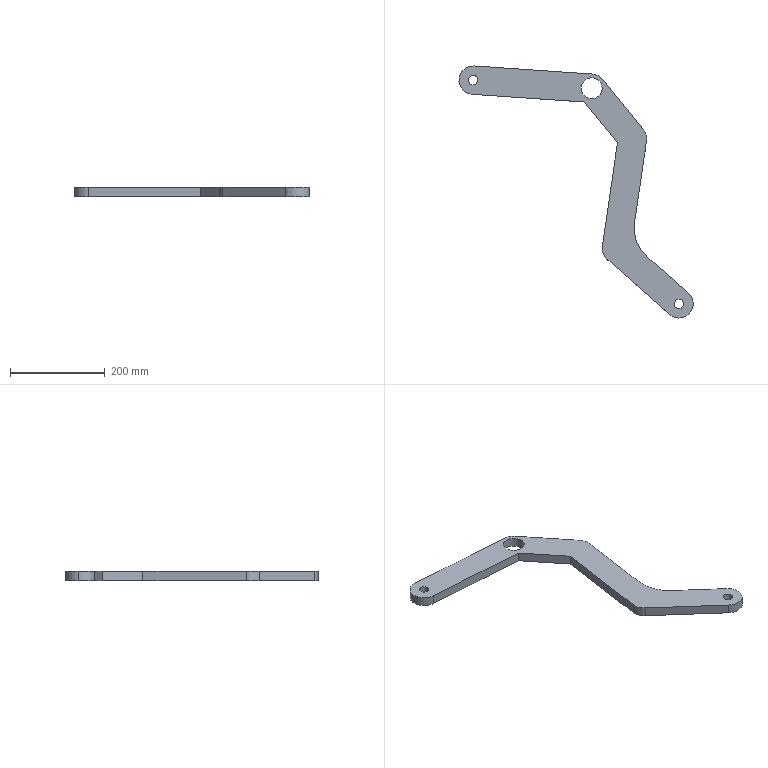Component | SolidWorks | IngotSupportRod-13 | 1 solid | 23 faces | box 494.09 x 531.83 x 20 mm | volume 974379 mm3 | cylinder 13 | plane 10 | commonest cylinder face diameters 60 x6 20 x4 44.189 x2 160 x1 | material 45
build123d program:
from build123d import *

# Parameters (mm, degrees)
SKETCH1_R           = 22.094
SKETCH1_R_2         = 10
BOSS_EXTRUDE1_DEPTH = 20
SKETCH2_R           = 22.094
BOSS_EXTRUDE2_DEPTH = 20
SKETCH3_R           = 10
CUT_EXTRUDE1_DEPTH  = 20


with BuildPart() as part:
    # Sketch1 → Boss-Extrude1 (new body)
    # profile 1 of 3: a face of its own
    with BuildSketch(Plane.XY):
        with BuildLine():
            Line((541.993, 526.894), (441.544, 620.054))
            ThreePointArc((441.544, 620.054), (399.148, 618.458), (400.744, 576.062))
            Line((400.744, 576.062), (491.593, 491.805))
            Line((491.593, 491.805), (491.593, 504.898))
            ThreePointArc((491.593, 504.898), (509.593, 532.394), (541.993, 526.894))
        make_face()
        with Locations((421.144, 598.058)):
            Circle(SKETCH1_R, mode=Mode.SUBTRACT)
    # profile 2 of 3: a face of its own
    with BuildSketch(Plane.XY):
        with BuildLine():
            Line((551.593, 330.656), (551.593, 504.898))
            ThreePointArc((551.593, 504.898), (533.593, 477.403), (501.193, 482.902))
            Line((501.193, 482.902), (491.593, 491.805))
            Line((491.593, 491.805), (491.593, 271.193))
            ThreePointArc((491.593, 271.193), (495.202, 256.927), (505.161, 246.094))
            Line((505.161, 246.094), (652.514, 149.626))
            ThreePointArc((652.514, 149.626), (694.046, 158.294), (685.378, 199.825))
            Line((685.378, 199.825), (587.775, 263.724))
            ThreePointArc((587.775, 263.724), (561.218, 292.613), (551.593, 330.656))
        make_face()
        with Locations((668.946, 174.726)):
            Circle(SKETCH1_R_2, mode=Mode.SUBTRACT)
    # profile 3 of 3: a face of its own
    with BuildSketch(Plane.XY):
        with BuildLine():
            ThreePointArc((551.593, 504.898), (549.089, 516.898), (541.993, 526.894))
            ThreePointArc((541.993, 526.894), (509.593, 532.394), (491.593, 504.898))
            Line((491.593, 504.898), (491.593, 491.805))
            Line((491.593, 491.805), (501.193, 482.902))
            ThreePointArc((501.193, 482.902), (533.593, 477.403), (551.593, 504.898))
        make_face()
    extrude(amount=BOSS_EXTRUDE1_DEPTH)

    # Sketch2 → Boss-Extrude2 (add)
    with BuildSketch(Plane.XY):
        with BuildLine():
            Line((423.445, 568.146), (173.493, 548.919))
            ThreePointArc((173.493, 548.919), (141.281, 576.53), (168.892, 608.742))
            Line((168.892, 608.742), (418.843, 627.97))
            ThreePointArc((418.843, 627.97), (451.056, 600.359), (423.445, 568.146))
        make_face()
        with Locations((421.144, 598.058)):
            Circle(SKETCH2_R, mode=Mode.SUBTRACT)
    extrude(amount=BOSS_EXTRUDE2_DEPTH)

    # Sketch3 → Cut-Extrude1 (cut)
    with BuildSketch(Plane.XY.offset(20)):
        with Locations((171.193, 578.831)):
            Circle(SKETCH3_R)
    extrude(amount=-CUT_EXTRUDE1_DEPTH, mode=Mode.SUBTRACT)


solid = part.part

# Placed as in the assembly
solid = solid.moved(Location((17.945, 67.185, 545), (0, 0, -8.314)))
STEP:
#1=COLOUR_RGB('',0.7922,0.8196,0.9333);
#2=FILL_AREA_STYLE_COLOUR('',#1);
#3=FILL_AREA_STYLE('',(#2));
#4=SURFACE_STYLE_FILL_AREA(#3);
#5=SURFACE_SIDE_STYLE('',(#4));
#6=SURFACE_STYLE_USAGE(.BOTH.,#5);
#7=PRESENTATION_STYLE_ASSIGNMENT((#6));
#8=CARTESIAN_POINT('',(10.281,24.276,21.457));
#9=VERTEX_POINT('',#8);
#10=CARTESIAN_POINT('',(11.06,24.163,21.457));
#11=VERTEX_POINT('',#10);
#12=CARTESIAN_POINT('',(10.671,24.22,21.457));
#13=DIRECTION('',(-0.,0.,1.));
#14=DIRECTION('',(0.9895,-0.1446,0.));
#15=AXIS2_PLACEMENT_3D('',#12,#13,#14);
#16=CIRCLE('',#15,0.3937);
#17=EDGE_CURVE('',#9,#11,#16,.T.);
#18=ORIENTED_EDGE('',*,*,#17,.F.);
#19=CARTESIAN_POINT('',(10.281,24.276,22.244));
#20=VERTEX_POINT('',#19);
#21=CARTESIAN_POINT('',(10.281,24.276,21.457));
#22=DIRECTION('',(-0.,0.,1.));
#23=VECTOR('',#22,39.37);
#24=LINE('',#21,#23);
#25=EDGE_CURVE('',#9,#20,#24,.T.);
#26=ORIENTED_EDGE('',*,*,#25,.T.);
#27=CARTESIAN_POINT('',(11.06,24.163,22.244));
#28=VERTEX_POINT('',#27);
#29=CARTESIAN_POINT('',(10.671,24.22,22.244));
#30=DIRECTION('',(-0.,0.,1.));
#31=DIRECTION('',(0.9895,-0.1446,0.));
#32=AXIS2_PLACEMENT_3D('',#29,#30,#31);
#33=CIRCLE('',#32,0.3937);
#34=EDGE_CURVE('',#20,#28,#33,.T.);
#35=ORIENTED_EDGE('',*,*,#34,.T.);
#36=CARTESIAN_POINT('',(11.06,24.163,21.457));
#37=DIRECTION('',(-0.,0.,1.));
#38=VECTOR('',#37,39.37);
#39=LINE('',#36,#38);
#40=EDGE_CURVE('',#11,#28,#39,.T.);
#41=ORIENTED_EDGE('',*,*,#40,.F.);
#42=EDGE_LOOP('',(#18,#26,#35,#41));
#43=FACE_OUTER_BOUND('',#42,.T.);
#44=CARTESIAN_POINT('',(10.671,24.22,21.457));
#45=DIRECTION('',(-0.,0.,1.));
#46=DIRECTION('',(0.9895,-0.1446,0.));
#47=AXIS2_PLACEMENT_3D('',#44,#45,#46);
#48=CYLINDRICAL_SURFACE('',#47,0.3937);
#49=ADVANCED_FACE('',(#43),#48,.F.);
#50=CARTESIAN_POINT('',(9.502,24.39,22.244));
#51=VERTEX_POINT('',#50);
#52=CARTESIAN_POINT('',(10.59,23.041,22.244));
#53=VERTEX_POINT('',#52);
#54=CARTESIAN_POINT('',(10.671,24.22,22.244));
#55=DIRECTION('',(-0.,0.,1.));
#56=DIRECTION('',(0.9895,-0.1446,0.));
#57=AXIS2_PLACEMENT_3D('',#54,#55,#56);
#58=CIRCLE('',#57,1.181);
#59=EDGE_CURVE('',#51,#53,#58,.T.);
#60=ORIENTED_EDGE('',*,*,#59,.F.);
#61=CARTESIAN_POINT('',(9.502,24.39,21.457));
#62=VERTEX_POINT('',#61);
#63=CARTESIAN_POINT('',(9.502,24.39,22.244));
#64=DIRECTION('',(0.,-0.,-1.));
#65=VECTOR('',#64,39.37);
#66=LINE('',#63,#65);
#67=EDGE_CURVE('',#51,#62,#66,.T.);
#68=ORIENTED_EDGE('',*,*,#67,.T.);
#69=CARTESIAN_POINT('',(10.59,23.041,21.457));
#70=VERTEX_POINT('',#69);
#71=CARTESIAN_POINT('',(10.671,24.22,21.457));
#72=DIRECTION('',(-0.,0.,1.));
#73=DIRECTION('',(0.9895,-0.1446,0.));
#74=AXIS2_PLACEMENT_3D('',#71,#72,#73);
#75=CIRCLE('',#74,1.181);
#76=EDGE_CURVE('',#62,#70,#75,.T.);
#77=ORIENTED_EDGE('',*,*,#76,.T.);
#78=CARTESIAN_POINT('',(10.59,23.041,22.244));
#79=DIRECTION('',(0.,-0.,-1.));
#80=VECTOR('',#79,39.37);
#81=LINE('',#78,#80);
#82=EDGE_CURVE('',#53,#70,#81,.T.);
#83=ORIENTED_EDGE('',*,*,#82,.F.);
#84=EDGE_LOOP('',(#60,#68,#77,#83));
#85=FACE_OUTER_BOUND('',#84,.T.);
#86=CARTESIAN_POINT('',(10.671,24.22,22.244));
#87=DIRECTION('',(0.,-0.,-1.));
#88=DIRECTION('',(-0.9895,0.1446,0.));
#89=AXIS2_PLACEMENT_3D('',#86,#87,#88);
#90=CYLINDRICAL_SURFACE('',#89,1.181);
#91=ADVANCED_FACE('',(#85),#90,.T.);
#92=CARTESIAN_POINT('',(27.371,5.7,22.244));
#93=VERTEX_POINT('',#92);
#94=CARTESIAN_POINT('',(28.15,5.586,22.244));
#95=VERTEX_POINT('',#94);
#96=CARTESIAN_POINT('',(27.761,5.643,22.244));
#97=DIRECTION('',(-0.,0.,1.));
#98=DIRECTION('',(0.9895,-0.1446,0.));
#99=AXIS2_PLACEMENT_3D('',#96,#97,#98);
#100=CIRCLE('',#99,0.3937);
#101=EDGE_CURVE('',#93,#95,#100,.T.);
#102=ORIENTED_EDGE('',*,*,#101,.T.);
#103=CARTESIAN_POINT('',(28.15,5.586,21.457));
#104=VERTEX_POINT('',#103);
#105=CARTESIAN_POINT('',(28.15,5.586,22.244));
#106=DIRECTION('',(0.,-0.,-1.));
#107=VECTOR('',#106,39.37);
#108=LINE('',#105,#107);
#109=EDGE_CURVE('',#95,#104,#108,.T.);
#110=ORIENTED_EDGE('',*,*,#109,.T.);
#111=CARTESIAN_POINT('',(27.371,5.7,21.457));
#112=VERTEX_POINT('',#111);
#113=CARTESIAN_POINT('',(27.761,5.643,21.457));
#114=DIRECTION('',(-0.,0.,1.));
#115=DIRECTION('',(0.9895,-0.1446,0.));
#116=AXIS2_PLACEMENT_3D('',#113,#114,#115);
#117=CIRCLE('',#116,0.3937);
#118=EDGE_CURVE('',#112,#104,#117,.T.);
#119=ORIENTED_EDGE('',*,*,#118,.F.);
#120=CARTESIAN_POINT('',(27.371,5.7,22.244));
#121=DIRECTION('',(0.,-0.,-1.));
#122=VECTOR('',#121,39.37);
#123=LINE('',#120,#122);
#124=EDGE_CURVE('',#93,#112,#123,.T.);
#125=ORIENTED_EDGE('',*,*,#124,.F.);
#126=EDGE_LOOP('',(#102,#110,#119,#125));
#127=FACE_OUTER_BOUND('',#126,.T.);
#128=CARTESIAN_POINT('',(27.761,5.643,22.244));
#129=DIRECTION('',(0.,-0.,-1.));
#130=DIRECTION('',(-0.9895,0.1446,0.));
#131=AXIS2_PLACEMENT_3D('',#128,#129,#130);
#132=CYLINDRICAL_SURFACE('',#131,0.3937);
#133=ADVANCED_FACE('',(#127),#132,.F.);
#134=CARTESIAN_POINT('',(19.657,23.671,22.244));
#135=VERTEX_POINT('',#134);
#136=CARTESIAN_POINT('',(21.378,23.42,22.244));
#137=VERTEX_POINT('',#136);
#138=CARTESIAN_POINT('',(20.517,23.546,22.244));
#139=DIRECTION('',(-0.,0.,1.));
#140=DIRECTION('',(0.9895,-0.1446,0.));
#141=AXIS2_PLACEMENT_3D('',#138,#139,#140);
#142=CIRCLE('',#141,0.8699);
#143=EDGE_CURVE('',#135,#137,#142,.T.);
#144=ORIENTED_EDGE('',*,*,#143,.T.);
#145=CARTESIAN_POINT('',(21.378,23.42,21.457));
#146=VERTEX_POINT('',#145);
#147=CARTESIAN_POINT('',(21.378,23.42,22.244));
#148=DIRECTION('',(0.,-0.,-1.));
#149=VECTOR('',#148,39.37);
#150=LINE('',#147,#149);
#151=EDGE_CURVE('',#137,#146,#150,.T.);
#152=ORIENTED_EDGE('',*,*,#151,.T.);
#153=CARTESIAN_POINT('',(19.657,23.671,21.457));
#154=VERTEX_POINT('',#153);
#155=CARTESIAN_POINT('',(20.517,23.546,21.457));
#156=DIRECTION('',(-0.,0.,1.));
#157=DIRECTION('',(0.9895,-0.1446,0.));
#158=AXIS2_PLACEMENT_3D('',#155,#156,#157);
#159=CIRCLE('',#158,0.8699);
#160=EDGE_CURVE('',#154,#146,#159,.T.);
#161=ORIENTED_EDGE('',*,*,#160,.F.);
#162=CARTESIAN_POINT('',(19.657,23.671,22.244));
#163=DIRECTION('',(0.,-0.,-1.));
#164=VECTOR('',#163,39.37);
#165=LINE('',#162,#164);
#166=EDGE_CURVE('',#135,#154,#165,.T.);
#167=ORIENTED_EDGE('',*,*,#166,.F.);
#168=EDGE_LOOP('',(#144,#152,#161,#167));
#169=FACE_OUTER_BOUND('',#168,.T.);
#170=CARTESIAN_POINT('',(20.517,23.546,22.244));
#171=DIRECTION('',(0.,-0.,-1.));
#172=DIRECTION('',(-0.9895,0.1446,0.));
#173=AXIS2_PLACEMENT_3D('',#170,#171,#172);
#174=CYLINDRICAL_SURFACE('',#173,0.8699);
#175=ADVANCED_FACE('',(#169),#174,.F.);
#176=CARTESIAN_POINT('',(20.598,24.724,22.244));
#177=VERTEX_POINT('',#176);
#178=CARTESIAN_POINT('',(20.598,24.724,21.457));
#179=VERTEX_POINT('',#178);
#180=CARTESIAN_POINT('',(20.598,24.724,22.244));
#181=DIRECTION('',(0.,-0.,-1.));
#182=VECTOR('',#181,39.37);
#183=LINE('',#180,#182);
#184=EDGE_CURVE('',#177,#179,#183,.T.);
#185=ORIENTED_EDGE('',*,*,#184,.F.);
#186=CARTESIAN_POINT('',(21.437,24.286,22.244));
#187=VERTEX_POINT('',#186);
#188=CARTESIAN_POINT('',(20.517,23.546,22.244));
#189=DIRECTION('',(-0.,0.,1.));
#190=DIRECTION('',(0.9895,-0.1446,0.));
#191=AXIS2_PLACEMENT_3D('',#188,#189,#190);
#192=CIRCLE('',#191,1.181);
#193=EDGE_CURVE('',#187,#177,#192,.T.);
#194=ORIENTED_EDGE('',*,*,#193,.F.);
#195=CARTESIAN_POINT('',(21.437,24.286,21.457));
#196=VERTEX_POINT('',#195);
#197=CARTESIAN_POINT('',(21.437,24.286,22.244));
#198=DIRECTION('',(0.,-0.,-1.));
#199=VECTOR('',#198,39.37);
#200=LINE('',#197,#199);
#201=EDGE_CURVE('',#187,#196,#200,.T.);
#202=ORIENTED_EDGE('',*,*,#201,.T.);
#203=CARTESIAN_POINT('',(20.517,23.546,21.457));
#204=DIRECTION('',(-0.,0.,1.));
#205=DIRECTION('',(0.9895,-0.1446,0.));
#206=AXIS2_PLACEMENT_3D('',#203,#204,#205);
#207=CIRCLE('',#206,1.181);
#208=EDGE_CURVE('',#196,#179,#207,.T.);
#209=ORIENTED_EDGE('',*,*,#208,.T.);
#210=EDGE_LOOP('',(#185,#194,#202,#209));
#211=FACE_OUTER_BOUND('',#210,.T.);
#212=CARTESIAN_POINT('',(20.517,23.546,22.244));
#213=DIRECTION('',(0.,-0.,-1.));
#214=DIRECTION('',(-0.9895,0.1446,0.));
#215=AXIS2_PLACEMENT_3D('',#212,#213,#214);
#216=CYLINDRICAL_SURFACE('',#215,1.181);
#217=ADVANCED_FACE('',(#211),#216,.T.);
#218=CARTESIAN_POINT('',(19.921,22.403,21.457));
#219=VERTEX_POINT('',#218);
#220=CARTESIAN_POINT('',(19.921,22.403,22.244));
#221=VERTEX_POINT('',#220);
#222=CARTESIAN_POINT('',(19.921,22.403,22.244));
#223=DIRECTION('',(-0.,0.,1.));
#224=VECTOR('',#223,39.37);
#225=LINE('',#222,#224);
#226=EDGE_CURVE('',#219,#221,#225,.T.);
#227=ORIENTED_EDGE('',*,*,#226,.F.);
#228=CARTESIAN_POINT('',(22.657,19.005,21.457));
#229=VERTEX_POINT('',#228);
#230=CARTESIAN_POINT('',(22.015,19.803,21.457));
#231=DIRECTION('',(0.6272,-0.7789,0.));
#232=VECTOR('',#231,39.37);
#233=LINE('',#230,#232);
#234=EDGE_CURVE('',#219,#229,#233,.T.);
#235=ORIENTED_EDGE('',*,*,#234,.T.);
#236=CARTESIAN_POINT('',(22.657,19.005,22.244));
#237=VERTEX_POINT('',#236);
#238=CARTESIAN_POINT('',(22.657,19.005,22.244));
#239=DIRECTION('',(0.,-0.,-1.));
#240=VECTOR('',#239,39.37);
#241=LINE('',#238,#240);
#242=EDGE_CURVE('',#237,#229,#241,.T.);
#243=ORIENTED_EDGE('',*,*,#242,.F.);
#244=CARTESIAN_POINT('',(22.015,19.803,22.244));
#245=DIRECTION('',(0.6272,-0.7789,0.));
#246=VECTOR('',#245,39.37);
#247=LINE('',#244,#246);
#248=EDGE_CURVE('',#221,#237,#247,.T.);
#249=ORIENTED_EDGE('',*,*,#248,.F.);
#250=EDGE_LOOP('',(#227,#235,#243,#249));
#251=FACE_OUTER_BOUND('',#250,.T.);
#252=CARTESIAN_POINT('',(22.015,19.803,22.244));
#253=DIRECTION('',(0.7789,0.6272,-0.));
#254=DIRECTION('',(-0.6272,0.7789,-0.));
#255=AXIS2_PLACEMENT_3D('',#252,#253,#254);
#256=PLANE('',#255);
#257=ADVANCED_FACE('',(#251),#256,.F.);
#258=CARTESIAN_POINT('',(25.069,19.174,21.457));
#259=VERTEX_POINT('',#258);
#260=CARTESIAN_POINT('',(24.077,12.386,21.457));
#261=VERTEX_POINT('',#260);
#262=CARTESIAN_POINT('',(22.195,-0.4952,21.457));
#263=DIRECTION('',(-0.1446,-0.9895,0.));
#264=VECTOR('',#263,39.37);
#265=LINE('',#262,#264);
#266=EDGE_CURVE('',#259,#261,#265,.T.);
#267=ORIENTED_EDGE('',*,*,#266,.F.);
#268=CARTESIAN_POINT('',(25.069,19.174,22.244));
#269=VERTEX_POINT('',#268);
#270=CARTESIAN_POINT('',(25.069,19.174,22.244));
#271=DIRECTION('',(0.,-0.,-1.));
#272=VECTOR('',#271,39.37);
#273=LINE('',#270,#272);
#274=EDGE_CURVE('',#269,#259,#273,.T.);
#275=ORIENTED_EDGE('',*,*,#274,.F.);
#276=CARTESIAN_POINT('',(24.077,12.386,22.244));
#277=VERTEX_POINT('',#276);
#278=CARTESIAN_POINT('',(22.195,-0.4952,22.244));
#279=DIRECTION('',(-0.1446,-0.9895,0.));
#280=VECTOR('',#279,39.37);
#281=LINE('',#278,#280);
#282=EDGE_CURVE('',#269,#277,#281,.T.);
#283=ORIENTED_EDGE('',*,*,#282,.T.);
#284=CARTESIAN_POINT('',(24.077,12.386,22.244));
#285=DIRECTION('',(0.,-0.,-1.));
#286=VECTOR('',#285,39.37);
#287=LINE('',#284,#286);
#288=EDGE_CURVE('',#277,#261,#287,.T.);
#289=ORIENTED_EDGE('',*,*,#288,.T.);
#290=EDGE_LOOP('',(#267,#275,#283,#289));
#291=FACE_OUTER_BOUND('',#290,.T.);
#292=CARTESIAN_POINT('',(22.195,-0.4952,22.244));
#293=DIRECTION('',(0.9895,-0.1446,0.));
#294=DIRECTION('',(0.,-0.,-1.));
#295=AXIS2_PLACEMENT_3D('',#292,#293,#294);
#296=PLANE('',#295);
#297=ADVANCED_FACE('',(#291),#296,.T.);
#298=CARTESIAN_POINT('',(24.82,20.085,21.457));
#299=VERTEX_POINT('',#298);
#300=CARTESIAN_POINT('',(23.9,19.345,21.457));
#301=DIRECTION('',(-0.,0.,1.));
#302=DIRECTION('',(0.9895,-0.1446,0.));
#303=AXIS2_PLACEMENT_3D('',#300,#301,#302);
#304=CIRCLE('',#303,1.181);
#305=EDGE_CURVE('',#259,#299,#304,.T.);
#306=ORIENTED_EDGE('',*,*,#305,.T.);
#307=CARTESIAN_POINT('',(24.82,20.085,22.244));
#308=VERTEX_POINT('',#307);
#309=CARTESIAN_POINT('',(24.82,20.085,22.244));
#310=DIRECTION('',(0.,-0.,-1.));
#311=VECTOR('',#310,39.37);
#312=LINE('',#309,#311);
#313=EDGE_CURVE('',#308,#299,#312,.T.);
#314=ORIENTED_EDGE('',*,*,#313,.F.);
#315=CARTESIAN_POINT('',(23.9,19.345,22.244));
#316=DIRECTION('',(-0.,0.,1.));
#317=DIRECTION('',(0.9895,-0.1446,0.));
#318=AXIS2_PLACEMENT_3D('',#315,#316,#317);
#319=CIRCLE('',#318,1.181);
#320=EDGE_CURVE('',#269,#308,#319,.T.);
#321=ORIENTED_EDGE('',*,*,#320,.F.);
#322=ORIENTED_EDGE('',*,*,#274,.T.);
#323=EDGE_LOOP('',(#306,#314,#321,#322));
#324=FACE_OUTER_BOUND('',#323,.T.);
#325=CARTESIAN_POINT('',(23.9,19.345,22.244));
#326=DIRECTION('',(0.,-0.,-1.));
#327=DIRECTION('',(-0.9895,0.1446,0.));
#328=AXIS2_PLACEMENT_3D('',#325,#326,#327);
#329=CYLINDRICAL_SURFACE('',#328,1.181);
#330=ADVANCED_FACE('',(#324),#329,.T.);
#331=CARTESIAN_POINT('',(23.855,21.284,21.457));
#332=DIRECTION('',(0.6272,-0.7789,0.));
#333=VECTOR('',#332,39.37);
#334=LINE('',#331,#333);
#335=EDGE_CURVE('',#196,#299,#334,.T.);
#336=ORIENTED_EDGE('',*,*,#335,.F.);
#337=ORIENTED_EDGE('',*,*,#201,.F.);
#338=CARTESIAN_POINT('',(23.855,21.284,22.244));
#339=DIRECTION('',(0.6272,-0.7789,0.));
#340=VECTOR('',#339,39.37);
#341=LINE('',#338,#340);
#342=EDGE_CURVE('',#187,#308,#341,.T.);
#343=ORIENTED_EDGE('',*,*,#342,.T.);
#344=ORIENTED_EDGE('',*,*,#313,.T.);
#345=EDGE_LOOP('',(#336,#337,#343,#344));
#346=FACE_OUTER_BOUND('',#345,.T.);
#347=CARTESIAN_POINT('',(23.855,21.284,22.244));
#348=DIRECTION('',(0.7789,0.6272,-0.));
#349=DIRECTION('',(-0.6272,0.7789,-0.));
#350=AXIS2_PLACEMENT_3D('',#347,#348,#349);
#351=PLANE('',#350);
#352=ADVANCED_FACE('',(#346),#351,.T.);
#353=CARTESIAN_POINT('',(21.401,10.411,21.457));
#354=VERTEX_POINT('',#353);
#355=CARTESIAN_POINT('',(19.857,-0.1536,21.457));
#356=DIRECTION('',(-0.1446,-0.9895,0.));
#357=VECTOR('',#356,39.37);
#358=LINE('',#355,#357);
#359=EDGE_CURVE('',#229,#354,#358,.T.);
#360=ORIENTED_EDGE('',*,*,#359,.T.);
#361=CARTESIAN_POINT('',(21.401,10.411,22.244));
#362=VERTEX_POINT('',#361);
#363=CARTESIAN_POINT('',(21.401,10.411,22.244));
#364=DIRECTION('',(0.,-0.,-1.));
#365=VECTOR('',#364,39.37);
#366=LINE('',#363,#365);
#367=EDGE_CURVE('',#362,#354,#366,.T.);
#368=ORIENTED_EDGE('',*,*,#367,.F.);
#369=CARTESIAN_POINT('',(19.857,-0.1536,22.244));
#370=DIRECTION('',(-0.1446,-0.9895,0.));
#371=VECTOR('',#370,39.37);
#372=LINE('',#369,#371);
#373=EDGE_CURVE('',#237,#362,#372,.T.);
#374=ORIENTED_EDGE('',*,*,#373,.F.);
#375=ORIENTED_EDGE('',*,*,#242,.T.);
#376=EDGE_LOOP('',(#360,#368,#374,#375));
#377=FACE_OUTER_BOUND('',#376,.T.);
#378=CARTESIAN_POINT('',(19.857,-0.1536,22.244));
#379=DIRECTION('',(0.9895,-0.1446,0.));
#380=DIRECTION('',(0.1446,0.9895,-0.));
#381=AXIS2_PLACEMENT_3D('',#378,#379,#380);
#382=PLANE('',#381);
#383=ADVANCED_FACE('',(#377),#382,.F.);
#384=CARTESIAN_POINT('',(21.787,9.356,21.457));
#385=VERTEX_POINT('',#384);
#386=CARTESIAN_POINT('',(22.57,10.24,21.457));
#387=DIRECTION('',(-0.,0.,1.));
#388=DIRECTION('',(0.9895,-0.1446,0.));
#389=AXIS2_PLACEMENT_3D('',#386,#387,#388);
#390=CIRCLE('',#389,1.181);
#391=EDGE_CURVE('',#354,#385,#390,.T.);
#392=ORIENTED_EDGE('',*,*,#391,.T.);
#393=CARTESIAN_POINT('',(21.787,9.356,22.244));
#394=VERTEX_POINT('',#393);
#395=CARTESIAN_POINT('',(21.787,9.356,22.244));
#396=DIRECTION('',(0.,-0.,-1.));
#397=VECTOR('',#396,39.37);
#398=LINE('',#395,#397);
#399=EDGE_CURVE('',#394,#385,#398,.T.);
#400=ORIENTED_EDGE('',*,*,#399,.F.);
#401=CARTESIAN_POINT('',(22.57,10.24,22.244));
#402=DIRECTION('',(-0.,0.,1.));
#403=DIRECTION('',(0.9895,-0.1446,0.));
#404=AXIS2_PLACEMENT_3D('',#401,#402,#403);
#405=CIRCLE('',#404,1.181);
#406=EDGE_CURVE('',#362,#394,#405,.T.);
#407=ORIENTED_EDGE('',*,*,#406,.F.);
#408=ORIENTED_EDGE('',*,*,#367,.T.);
#409=EDGE_LOOP('',(#392,#400,#407,#408));
#410=FACE_OUTER_BOUND('',#409,.T.);
#411=CARTESIAN_POINT('',(22.57,10.24,22.244));
#412=DIRECTION('',(0.,-0.,-1.));
#413=DIRECTION('',(-0.9895,0.1446,0.));
#414=AXIS2_PLACEMENT_3D('',#411,#412,#413);
#415=CYLINDRICAL_SURFACE('',#414,1.181);
#416=ADVANCED_FACE('',(#410),#415,.T.);
#417=CARTESIAN_POINT('',(26.978,4.759,21.457));
#418=VERTEX_POINT('',#417);
#419=CARTESIAN_POINT('',(13.302,16.869,21.457));
#420=DIRECTION('',(0.7487,-0.663,0.));
#421=VECTOR('',#420,39.37);
#422=LINE('',#419,#421);
#423=EDGE_CURVE('',#385,#418,#422,.T.);
#424=ORIENTED_EDGE('',*,*,#423,.T.);
#425=CARTESIAN_POINT('',(26.978,4.759,22.244));
#426=VERTEX_POINT('',#425);
#427=CARTESIAN_POINT('',(26.978,4.759,22.244));
#428=DIRECTION('',(0.,-0.,-1.));
#429=VECTOR('',#428,39.37);
#430=LINE('',#427,#429);
#431=EDGE_CURVE('',#426,#418,#430,.T.);
#432=ORIENTED_EDGE('',*,*,#431,.F.);
#433=CARTESIAN_POINT('',(13.302,16.869,22.244));
#434=DIRECTION('',(0.7487,-0.663,0.));
#435=VECTOR('',#434,39.37);
#436=LINE('',#433,#435);
#437=EDGE_CURVE('',#394,#426,#436,.T.);
#438=ORIENTED_EDGE('',*,*,#437,.F.);
#439=ORIENTED_EDGE('',*,*,#399,.T.);
#440=EDGE_LOOP('',(#424,#432,#438,#439));
#441=FACE_OUTER_BOUND('',#440,.T.);
#442=CARTESIAN_POINT('',(13.302,16.869,22.244));
#443=DIRECTION('',(0.663,0.7487,-0.));
#444=DIRECTION('',(-0.7487,0.663,-0.));
#445=AXIS2_PLACEMENT_3D('',#442,#443,#444);
#446=PLANE('',#445);
#447=ADVANCED_FACE('',(#441),#446,.F.);
#448=CARTESIAN_POINT('',(28.544,6.528,21.457));
#449=VERTEX_POINT('',#448);
#450=CARTESIAN_POINT('',(27.761,5.643,21.457));
#451=DIRECTION('',(-0.,0.,1.));
#452=DIRECTION('',(0.9895,-0.1446,0.));
#453=AXIS2_PLACEMENT_3D('',#450,#451,#452);
#454=CIRCLE('',#453,1.181);
#455=EDGE_CURVE('',#418,#449,#454,.T.);
#456=ORIENTED_EDGE('',*,*,#455,.T.);
#457=CARTESIAN_POINT('',(28.544,6.528,22.244));
#458=VERTEX_POINT('',#457);
#459=CARTESIAN_POINT('',(28.544,6.528,22.244));
#460=DIRECTION('',(0.,-0.,-1.));
#461=VECTOR('',#460,39.37);
#462=LINE('',#459,#461);
#463=EDGE_CURVE('',#458,#449,#462,.T.);
#464=ORIENTED_EDGE('',*,*,#463,.F.);
#465=CARTESIAN_POINT('',(27.761,5.643,22.244));
#466=DIRECTION('',(-0.,0.,1.));
#467=DIRECTION('',(0.9895,-0.1446,0.));
#468=AXIS2_PLACEMENT_3D('',#465,#466,#467);
#469=CIRCLE('',#468,1.181);
#470=EDGE_CURVE('',#426,#458,#469,.T.);
#471=ORIENTED_EDGE('',*,*,#470,.F.);
#472=ORIENTED_EDGE('',*,*,#431,.T.);
#473=EDGE_LOOP('',(#456,#464,#471,#472));
#474=FACE_OUTER_BOUND('',#473,.T.);
#475=CARTESIAN_POINT('',(27.761,5.643,22.244));
#476=DIRECTION('',(0.,-0.,-1.));
#477=DIRECTION('',(-0.9895,0.1446,0.));
#478=AXIS2_PLACEMENT_3D('',#475,#476,#477);
#479=CYLINDRICAL_SURFACE('',#478,1.181);
#480=ADVANCED_FACE('',(#474),#479,.T.);
#481=CARTESIAN_POINT('',(25.105,9.573,21.457));
#482=VERTEX_POINT('',#481);
#483=CARTESIAN_POINT('',(14.868,18.638,21.457));
#484=DIRECTION('',(0.7487,-0.663,0.));
#485=VECTOR('',#484,39.37);
#486=LINE('',#483,#485);
#487=EDGE_CURVE('',#482,#449,#486,.T.);
#488=ORIENTED_EDGE('',*,*,#487,.F.);
#489=CARTESIAN_POINT('',(25.105,9.573,22.244));
#490=VERTEX_POINT('',#489);
#491=CARTESIAN_POINT('',(25.105,9.573,22.244));
#492=DIRECTION('',(0.,-0.,-1.));
#493=VECTOR('',#492,39.37);
#494=LINE('',#491,#493);
#495=EDGE_CURVE('',#490,#482,#494,.T.);
#496=ORIENTED_EDGE('',*,*,#495,.F.);
#497=CARTESIAN_POINT('',(14.868,18.638,22.244));
#498=DIRECTION('',(0.7487,-0.663,0.));
#499=VECTOR('',#498,39.37);
#500=LINE('',#497,#499);
#501=EDGE_CURVE('',#490,#458,#500,.T.);
#502=ORIENTED_EDGE('',*,*,#501,.T.);
#503=ORIENTED_EDGE('',*,*,#463,.T.);
#504=EDGE_LOOP('',(#488,#496,#502,#503));
#505=FACE_OUTER_BOUND('',#504,.T.);
#506=CARTESIAN_POINT('',(14.868,18.638,22.244));
#507=DIRECTION('',(0.663,0.7487,-0.));
#508=DIRECTION('',(-0.7487,0.663,-0.));
#509=AXIS2_PLACEMENT_3D('',#506,#507,#508);
#510=PLANE('',#509);
#511=ADVANCED_FACE('',(#505),#510,.T.);
#512=ORIENTED_EDGE('',*,*,#151,.F.);
#513=CARTESIAN_POINT('',(20.517,23.546,22.244));
#514=DIRECTION('',(-0.,0.,1.));
#515=DIRECTION('',(0.9895,-0.1446,0.));
#516=AXIS2_PLACEMENT_3D('',#513,#514,#515);
#517=CIRCLE('',#516,0.8699);
#518=EDGE_CURVE('',#137,#135,#517,.T.);
#519=ORIENTED_EDGE('',*,*,#518,.T.);
#520=ORIENTED_EDGE('',*,*,#166,.T.);
#521=CARTESIAN_POINT('',(20.517,23.546,21.457));
#522=DIRECTION('',(-0.,0.,1.));
#523=DIRECTION('',(0.9895,-0.1446,0.));
#524=AXIS2_PLACEMENT_3D('',#521,#522,#523);
#525=CIRCLE('',#524,0.8699);
#526=EDGE_CURVE('',#146,#154,#525,.T.);
#527=ORIENTED_EDGE('',*,*,#526,.F.);
#528=EDGE_LOOP('',(#512,#519,#520,#527));
#529=FACE_OUTER_BOUND('',#528,.T.);
#530=CARTESIAN_POINT('',(20.517,23.546,22.244));
#531=DIRECTION('',(0.,-0.,-1.));
#532=DIRECTION('',(-0.9895,0.1446,0.));
#533=AXIS2_PLACEMENT_3D('',#530,#531,#532);
#534=CYLINDRICAL_SURFACE('',#533,0.8699);
#535=ADVANCED_FACE('',(#529),#534,.F.);
#536=CARTESIAN_POINT('',(27.193,11.93,21.457));
#537=DIRECTION('',(0.,-0.,-1.));
#538=DIRECTION('',(0.9895,-0.1446,0.));
#539=AXIS2_PLACEMENT_3D('',#536,#537,#538);
#540=CIRCLE('',#539,3.15);
#541=EDGE_CURVE('',#482,#261,#540,.T.);
#542=ORIENTED_EDGE('',*,*,#541,.T.);
#543=ORIENTED_EDGE('',*,*,#288,.F.);
#544=CARTESIAN_POINT('',(27.193,11.93,22.244));
#545=DIRECTION('',(0.,-0.,-1.));
#546=DIRECTION('',(0.9895,-0.1446,0.));
#547=AXIS2_PLACEMENT_3D('',#544,#545,#546);
#548=CIRCLE('',#547,3.15);
#549=EDGE_CURVE('',#490,#277,#548,.T.);
#550=ORIENTED_EDGE('',*,*,#549,.F.);
#551=ORIENTED_EDGE('',*,*,#495,.T.);
#552=EDGE_LOOP('',(#542,#543,#550,#551));
#553=FACE_OUTER_BOUND('',#552,.T.);
#554=CARTESIAN_POINT('',(27.193,11.93,22.244));
#555=DIRECTION('',(0.,-0.,-1.));
#556=DIRECTION('',(-0.9895,0.1446,0.));
#557=AXIS2_PLACEMENT_3D('',#554,#555,#556);
#558=CYLINDRICAL_SURFACE('',#557,3.15);
#559=ADVANCED_FACE('',(#553),#558,.F.);
#560=ORIENTED_EDGE('',*,*,#109,.F.);
#561=CARTESIAN_POINT('',(27.761,5.643,22.244));
#562=DIRECTION('',(-0.,0.,1.));
#563=DIRECTION('',(0.9895,-0.1446,0.));
#564=AXIS2_PLACEMENT_3D('',#561,#562,#563);
#565=CIRCLE('',#564,0.3937);
#566=EDGE_CURVE('',#95,#93,#565,.T.);
#567=ORIENTED_EDGE('',*,*,#566,.T.);
#568=ORIENTED_EDGE('',*,*,#124,.T.);
#569=CARTESIAN_POINT('',(27.761,5.643,21.457));
#570=DIRECTION('',(-0.,0.,1.));
#571=DIRECTION('',(0.9895,-0.1446,0.));
#572=AXIS2_PLACEMENT_3D('',#569,#570,#571);
#573=CIRCLE('',#572,0.3937);
#574=EDGE_CURVE('',#104,#112,#573,.T.);
#575=ORIENTED_EDGE('',*,*,#574,.F.);
#576=EDGE_LOOP('',(#560,#567,#568,#575));
#577=FACE_OUTER_BOUND('',#576,.T.);
#578=CARTESIAN_POINT('',(27.761,5.643,22.244));
#579=DIRECTION('',(0.,-0.,-1.));
#580=DIRECTION('',(-0.9895,0.1446,0.));
#581=AXIS2_PLACEMENT_3D('',#578,#579,#580);
#582=CYLINDRICAL_SURFACE('',#581,0.3937);
#583=ADVANCED_FACE('',(#577),#582,.F.);
#584=CARTESIAN_POINT('',(10.671,24.22,22.244));
#585=DIRECTION('',(-0.,0.,1.));
#586=DIRECTION('',(0.9895,-0.1446,0.));
#587=AXIS2_PLACEMENT_3D('',#584,#585,#586);
#588=CIRCLE('',#587,0.3937);
#589=EDGE_CURVE('',#28,#20,#588,.T.);
#590=ORIENTED_EDGE('',*,*,#589,.F.);
#591=ORIENTED_EDGE('',*,*,#34,.F.);
#592=EDGE_LOOP('',(#590,#591));
#593=FACE_BOUND('',#592,.T.);
#594=ORIENTED_EDGE('',*,*,#342,.F.);
#595=ORIENTED_EDGE('',*,*,#193,.T.);
#596=CARTESIAN_POINT('',(10.751,25.398,22.244));
#597=VERTEX_POINT('',#596);
#598=CARTESIAN_POINT('',(20.598,24.724,22.244));
#599=DIRECTION('',(-0.9977,0.06829,-0.));
#600=VECTOR('',#599,39.37);
#601=LINE('',#598,#600);
#602=EDGE_CURVE('',#177,#597,#601,.T.);
#603=ORIENTED_EDGE('',*,*,#602,.T.);
#604=CARTESIAN_POINT('',(10.671,24.22,22.244));
#605=DIRECTION('',(-0.,0.,1.));
#606=DIRECTION('',(0.9895,-0.1446,0.));
#607=AXIS2_PLACEMENT_3D('',#604,#605,#606);
#608=CIRCLE('',#607,1.181);
#609=EDGE_CURVE('',#597,#51,#608,.T.);
#610=ORIENTED_EDGE('',*,*,#609,.T.);
#611=ORIENTED_EDGE('',*,*,#59,.T.);
#612=CARTESIAN_POINT('',(20.437,22.367,22.244));
#613=DIRECTION('',(0.9977,-0.06829,0.));
#614=VECTOR('',#613,39.37);
#615=LINE('',#612,#614);
#616=EDGE_CURVE('',#53,#221,#615,.T.);
#617=ORIENTED_EDGE('',*,*,#616,.T.);
#618=ORIENTED_EDGE('',*,*,#248,.T.);
#619=ORIENTED_EDGE('',*,*,#373,.T.);
#620=ORIENTED_EDGE('',*,*,#406,.T.);
#621=ORIENTED_EDGE('',*,*,#437,.T.);
#622=ORIENTED_EDGE('',*,*,#470,.T.);
#623=ORIENTED_EDGE('',*,*,#501,.F.);
#624=ORIENTED_EDGE('',*,*,#549,.T.);
#625=ORIENTED_EDGE('',*,*,#282,.F.);
#626=ORIENTED_EDGE('',*,*,#320,.T.);
#627=EDGE_LOOP('',(#594,#595,#603,#610,#611,#617,#618,#619,#620,#621,#622,#623,#624,#625,#626));
#628=FACE_OUTER_BOUND('',#627,.T.);
#629=ORIENTED_EDGE('',*,*,#143,.F.);
#630=ORIENTED_EDGE('',*,*,#518,.F.);
#631=EDGE_LOOP('',(#629,#630));
#632=FACE_BOUND('',#631,.T.);
#633=ORIENTED_EDGE('',*,*,#101,.F.);
#634=ORIENTED_EDGE('',*,*,#566,.F.);
#635=EDGE_LOOP('',(#633,#634));
#636=FACE_BOUND('',#635,.T.);
#637=CARTESIAN_POINT('',(0.7065,2.645,22.244));
#638=DIRECTION('',(-0.,0.,1.));
#639=DIRECTION('',(0.9895,-0.1446,0.));
#640=AXIS2_PLACEMENT_3D('',#637,#638,#639);
#641=PLANE('',#640);
#642=ADVANCED_FACE('',(#593,#628,#632,#636),#641,.T.);
#643=CARTESIAN_POINT('',(10.671,24.22,21.457));
#644=DIRECTION('',(-0.,0.,1.));
#645=DIRECTION('',(0.9895,-0.1446,0.));
#646=AXIS2_PLACEMENT_3D('',#643,#644,#645);
#647=CIRCLE('',#646,0.3937);
#648=EDGE_CURVE('',#11,#9,#647,.T.);
#649=ORIENTED_EDGE('',*,*,#648,.T.);
#650=ORIENTED_EDGE('',*,*,#17,.T.);
#651=EDGE_LOOP('',(#649,#650));
#652=FACE_BOUND('',#651,.T.);
#653=ORIENTED_EDGE('',*,*,#208,.F.);
#654=ORIENTED_EDGE('',*,*,#335,.T.);
#655=ORIENTED_EDGE('',*,*,#305,.F.);
#656=ORIENTED_EDGE('',*,*,#266,.T.);
#657=ORIENTED_EDGE('',*,*,#541,.F.);
#658=ORIENTED_EDGE('',*,*,#487,.T.);
#659=ORIENTED_EDGE('',*,*,#455,.F.);
#660=ORIENTED_EDGE('',*,*,#423,.F.);
#661=ORIENTED_EDGE('',*,*,#391,.F.);
#662=ORIENTED_EDGE('',*,*,#359,.F.);
#663=ORIENTED_EDGE('',*,*,#234,.F.);
#664=CARTESIAN_POINT('',(20.437,22.367,21.457));
#665=DIRECTION('',(0.9977,-0.06829,0.));
#666=VECTOR('',#665,39.37);
#667=LINE('',#664,#666);
#668=EDGE_CURVE('',#70,#219,#667,.T.);
#669=ORIENTED_EDGE('',*,*,#668,.F.);
#670=ORIENTED_EDGE('',*,*,#76,.F.);
#671=CARTESIAN_POINT('',(10.751,25.398,21.457));
#672=VERTEX_POINT('',#671);
#673=CARTESIAN_POINT('',(10.671,24.22,21.457));
#674=DIRECTION('',(-0.,0.,1.));
#675=DIRECTION('',(0.9895,-0.1446,0.));
#676=AXIS2_PLACEMENT_3D('',#673,#674,#675);
#677=CIRCLE('',#676,1.181);
#678=EDGE_CURVE('',#672,#62,#677,.T.);
#679=ORIENTED_EDGE('',*,*,#678,.F.);
#680=CARTESIAN_POINT('',(20.598,24.724,21.457));
#681=DIRECTION('',(-0.9977,0.06829,-0.));
#682=VECTOR('',#681,39.37);
#683=LINE('',#680,#682);
#684=EDGE_CURVE('',#179,#672,#683,.T.);
#685=ORIENTED_EDGE('',*,*,#684,.F.);
#686=EDGE_LOOP('',(#653,#654,#655,#656,#657,#658,#659,#660,#661,#662,#663,#669,#670,#679,#685));
#687=FACE_OUTER_BOUND('',#686,.T.);
#688=ORIENTED_EDGE('',*,*,#160,.T.);
#689=ORIENTED_EDGE('',*,*,#526,.T.);
#690=EDGE_LOOP('',(#688,#689));
#691=FACE_BOUND('',#690,.T.);
#692=ORIENTED_EDGE('',*,*,#118,.T.);
#693=ORIENTED_EDGE('',*,*,#574,.T.);
#694=EDGE_LOOP('',(#692,#693));
#695=FACE_BOUND('',#694,.T.);
#696=CARTESIAN_POINT('',(0.7065,2.645,21.457));
#697=DIRECTION('',(-0.,0.,1.));
#698=DIRECTION('',(0.9895,-0.1446,0.));
#699=AXIS2_PLACEMENT_3D('',#696,#697,#698);
#700=PLANE('',#699);
#701=ADVANCED_FACE('',(#652,#687,#691,#695),#700,.F.);
#702=ORIENTED_EDGE('',*,*,#668,.T.);
#703=ORIENTED_EDGE('',*,*,#226,.T.);
#704=ORIENTED_EDGE('',*,*,#616,.F.);
#705=ORIENTED_EDGE('',*,*,#82,.T.);
#706=EDGE_LOOP('',(#702,#703,#704,#705));
#707=FACE_OUTER_BOUND('',#706,.T.);
#708=CARTESIAN_POINT('',(20.437,22.367,22.244));
#709=DIRECTION('',(0.06829,0.9977,-0.));
#710=DIRECTION('',(-0.9977,0.06829,-0.));
#711=AXIS2_PLACEMENT_3D('',#708,#709,#710);
#712=PLANE('',#711);
#713=ADVANCED_FACE('',(#707),#712,.F.);
#714=ORIENTED_EDGE('',*,*,#684,.T.);
#715=CARTESIAN_POINT('',(10.751,25.398,22.244));
#716=DIRECTION('',(0.,-0.,-1.));
#717=VECTOR('',#716,39.37);
#718=LINE('',#715,#717);
#719=EDGE_CURVE('',#597,#672,#718,.T.);
#720=ORIENTED_EDGE('',*,*,#719,.F.);
#721=ORIENTED_EDGE('',*,*,#602,.F.);
#722=ORIENTED_EDGE('',*,*,#184,.T.);
#723=EDGE_LOOP('',(#714,#720,#721,#722));
#724=FACE_OUTER_BOUND('',#723,.T.);
#725=CARTESIAN_POINT('',(20.598,24.724,22.244));
#726=DIRECTION('',(-0.06829,-0.9977,0.));
#727=DIRECTION('',(0.9977,-0.06829,0.));
#728=AXIS2_PLACEMENT_3D('',#725,#726,#727);
#729=PLANE('',#728);
#730=ADVANCED_FACE('',(#724),#729,.F.);
#731=ORIENTED_EDGE('',*,*,#67,.F.);
#732=ORIENTED_EDGE('',*,*,#609,.F.);
#733=ORIENTED_EDGE('',*,*,#719,.T.);
#734=ORIENTED_EDGE('',*,*,#678,.T.);
#735=EDGE_LOOP('',(#731,#732,#733,#734));
#736=FACE_OUTER_BOUND('',#735,.T.);
#737=CARTESIAN_POINT('',(10.671,24.22,22.244));
#738=DIRECTION('',(0.,-0.,-1.));
#739=DIRECTION('',(-0.9895,0.1446,0.));
#740=AXIS2_PLACEMENT_3D('',#737,#738,#739);
#741=CYLINDRICAL_SURFACE('',#740,1.181);
#742=ADVANCED_FACE('',(#736),#741,.T.);
#743=ORIENTED_EDGE('',*,*,#25,.F.);
#744=ORIENTED_EDGE('',*,*,#648,.F.);
#745=ORIENTED_EDGE('',*,*,#40,.T.);
#746=ORIENTED_EDGE('',*,*,#589,.T.);
#747=EDGE_LOOP('',(#743,#744,#745,#746));
#748=FACE_OUTER_BOUND('',#747,.T.);
#749=CARTESIAN_POINT('',(10.671,24.22,21.457));
#750=DIRECTION('',(-0.,0.,1.));
#751=DIRECTION('',(0.9895,-0.1446,0.));
#752=AXIS2_PLACEMENT_3D('',#749,#750,#751);
#753=CYLINDRICAL_SURFACE('',#752,0.3937);
#754=ADVANCED_FACE('',(#748),#753,.F.);
#755=CLOSED_SHELL('',(#49,#91,#133,#175,#217,#257,#297,#330,#352,#383,#416,#447,#480,#511,#535,#559,#583,#642,#701,#713,#730,#742,#754));
#756=MANIFOLD_SOLID_BREP('',#755);
#757=STYLED_ITEM('',(#7),#756);
#758=(LENGTH_UNIT()NAMED_UNIT(*)SI_UNIT($,.METRE.));
#759=LENGTH_MEASURE_WITH_UNIT(LENGTH_MEASURE(0.0254),#758);
#760=DIMENSIONAL_EXPONENTS(1.,0.,0.,0.,0.,0.,0.);
#761=(CONVERSION_BASED_UNIT('',#759)LENGTH_UNIT()NAMED_UNIT(#760));
#762=UNCERTAINTY_MEASURE_WITH_UNIT(LENGTH_MEASURE(0.00001),#761,'','');
#763=(NAMED_UNIT(*)PLANE_ANGLE_UNIT()SI_UNIT($,.RADIAN.));
#764=(NAMED_UNIT(*)SI_UNIT($,.STERADIAN.)SOLID_ANGLE_UNIT());
#765=(GEOMETRIC_REPRESENTATION_CONTEXT(3)GLOBAL_UNCERTAINTY_ASSIGNED_CONTEXT((#762))GLOBAL_UNIT_ASSIGNED_CONTEXT((#761,#763,#764))REPRESENTATION_CONTEXT('',''));
#766=MECHANICAL_DESIGN_GEOMETRIC_PRESENTATION_REPRESENTATION('',(#757),#765);
#767=CARTESIAN_POINT('',(0.,0.,0.));
#768=DIRECTION('',(0.,0.,1.));
#769=DIRECTION('',(1.,0.,0.));
#770=AXIS2_PLACEMENT_3D('',#767,#768,#769);
#771=(LENGTH_UNIT()NAMED_UNIT(*)SI_UNIT($,.METRE.));
#772=LENGTH_MEASURE_WITH_UNIT(LENGTH_MEASURE(0.0254),#771);
#773=DIMENSIONAL_EXPONENTS(1.,0.,0.,0.,0.,0.,0.);
#774=(CONVERSION_BASED_UNIT('',#772)LENGTH_UNIT()NAMED_UNIT(#773));
#775=UNCERTAINTY_MEASURE_WITH_UNIT(LENGTH_MEASURE(0.00001),#774,'','');
#776=(NAMED_UNIT(*)PLANE_ANGLE_UNIT()SI_UNIT($,.RADIAN.));
#777=(NAMED_UNIT(*)SI_UNIT($,.STERADIAN.)SOLID_ANGLE_UNIT());
#778=(GEOMETRIC_REPRESENTATION_CONTEXT(3)GLOBAL_UNCERTAINTY_ASSIGNED_CONTEXT((#775))GLOBAL_UNIT_ASSIGNED_CONTEXT((#774,#776,#777))REPRESENTATION_CONTEXT('',''));
#779=ADVANCED_BREP_SHAPE_REPRESENTATION('',(#756,#770),#778);
#780=PRESENTATION_LAYER_ASSIGNMENT('','',(#757));